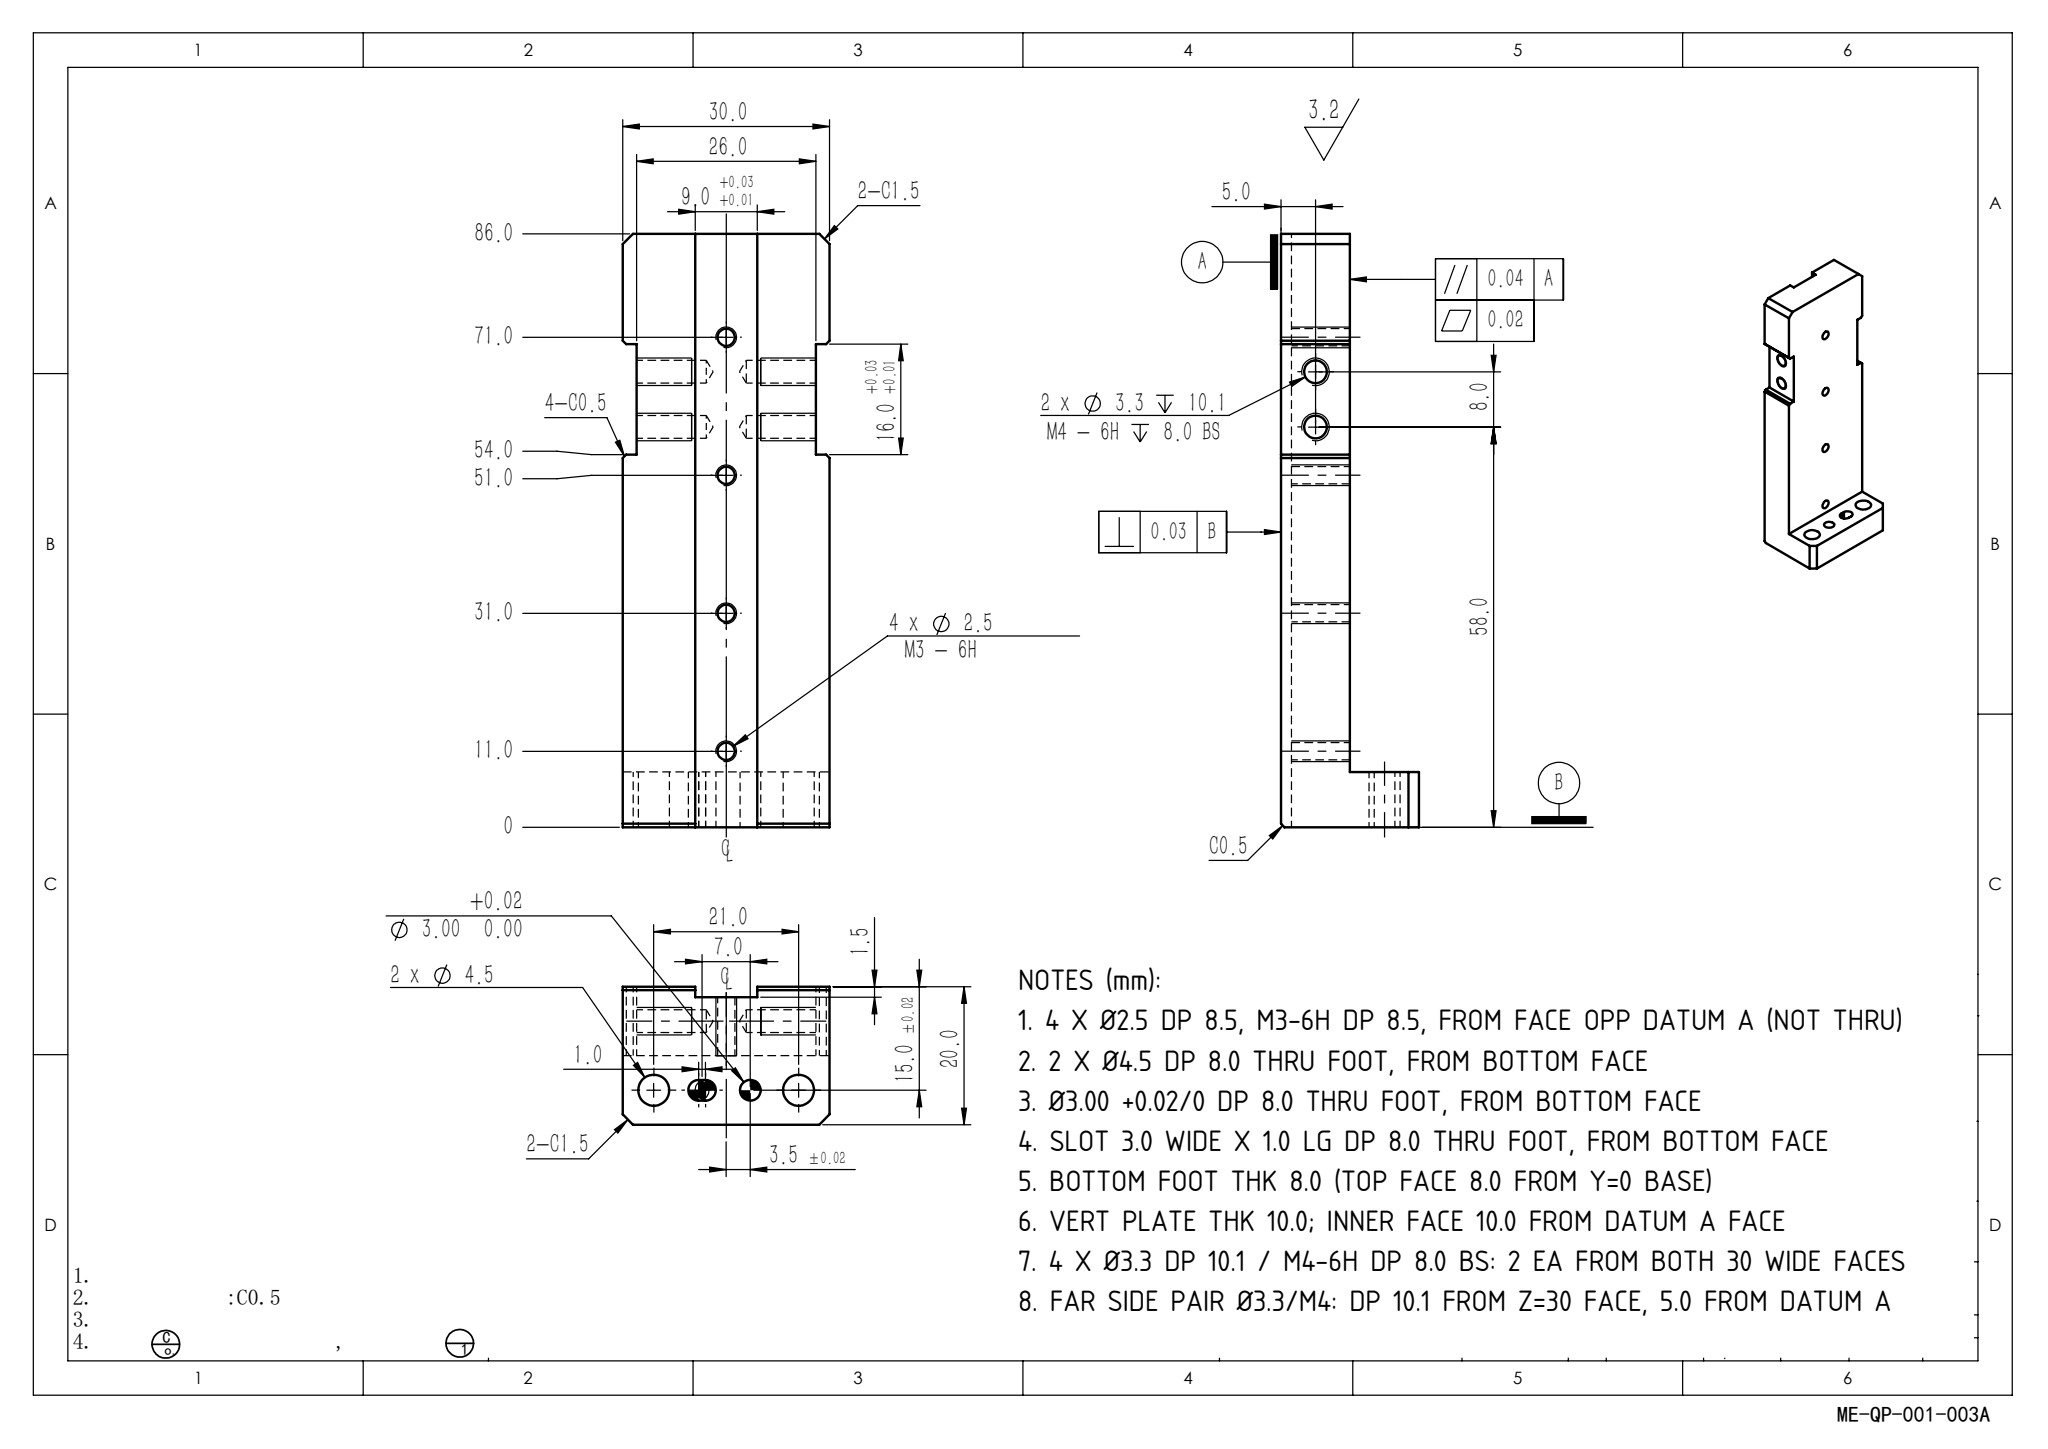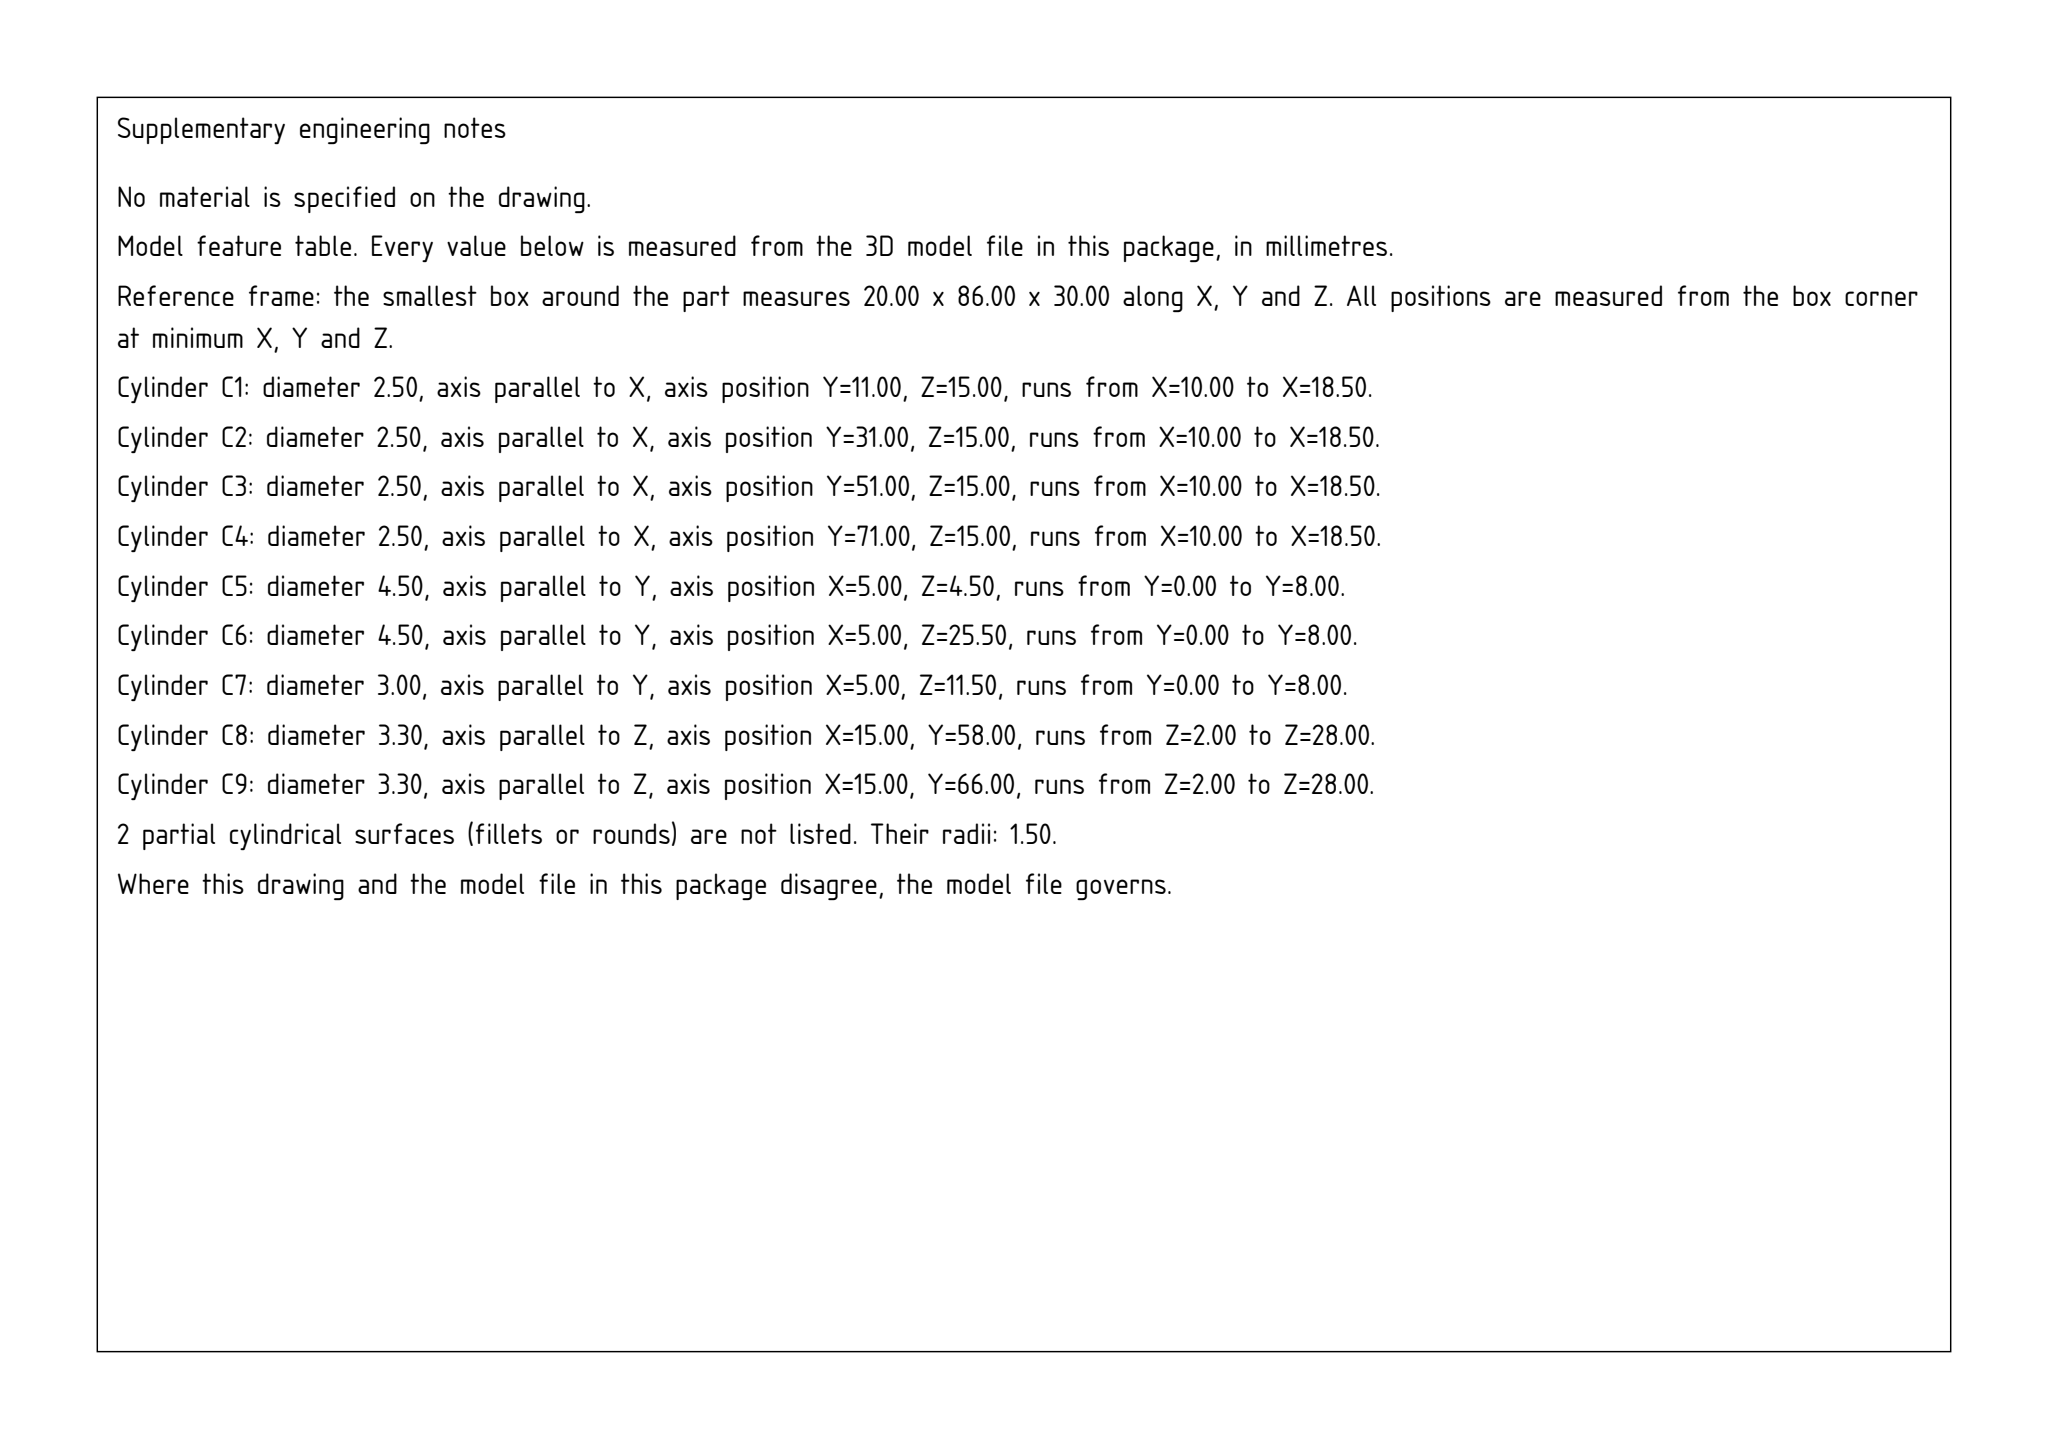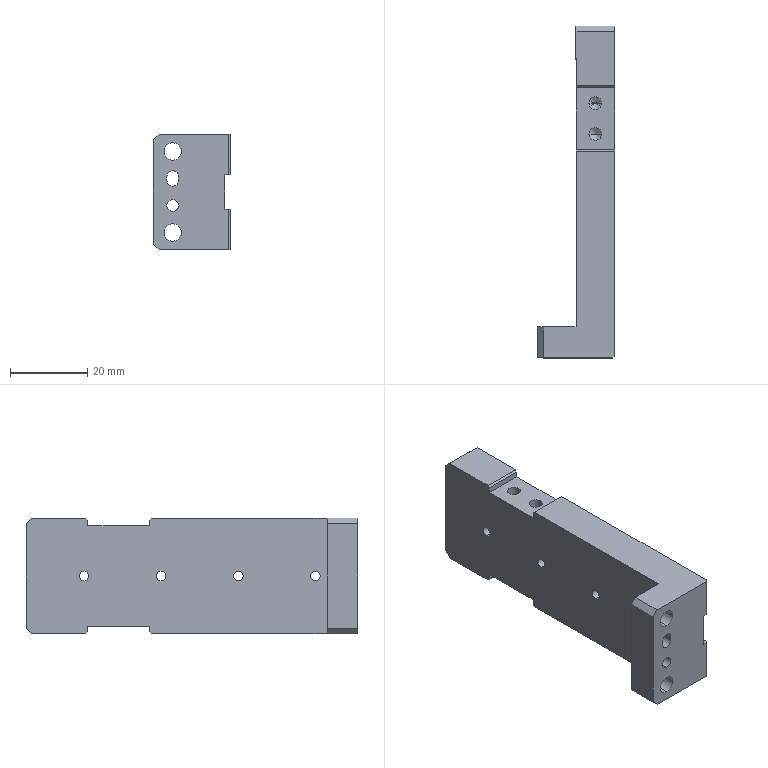Part | SolidWorks | mm | 1 solid | 64 faces | box 20 x 86 x 30 mm | volume 25436 mm3 | plane 32 | cylinder 24 | cone 8 | commonest cylinder face diameters 3.3 x8 2.5 x8 3 x4 4.5 x4
Drawing notes:
4 X Ø2.5 DP 8.5, M3-6H DP 8.5, FROM FACE OPP DATUM A (NOT THRU) | from the solid: cyl dia2.5 axis x len 8.5 at y=11/31/51/71, z=15; faces x=10.0 to x=18.5
2 X Ø4.5 DP 8.0 THRU FOOT, FROM BOTTOM FACE | from the solid: cyl dia4.5 axis y len 8.0 at x=5.0, z=4.5 & 25.5; foot face y=0 to 8.0
Ø3.00 +0.02/0 DP 8.0 THRU FOOT, FROM BOTTOM FACE | from the solid: cyl dia3.0 axis y len 8.0 at x=5.0, z=11.5
SLOT 3.0 WIDE X 1.0 LG DP 8.0 THRU FOOT, FROM BOTTOM FACE | from the solid: cyl dia3.0 axis y len 8.0 at z=18.0 & 19.0, x=5.0
BOTTOM FOOT THK 8.0 (TOP FACE 8.0 FROM Y=0 BASE) | from the solid: planes y=0.0 and y=8.0
VERT PLATE THK 10.0; INNER FACE 10.0 FROM DATUM A FACE | from the solid: planes x=20.0 (datum A) and x=10.0; overall 20.0
4 X Ø3.3 DP 10.1 / M4-6H DP 8.0 BS: 2 EA FROM BOTH 30 WIDE FACES | from the solid: dia3.3 axis z len 10.1 at (x=15, y=58) & (x=15, y=66), 4 off
FAR SIDE PAIR Ø3.3/M4: DP 10.1 FROM Z=30 FACE, 5.0 FROM DATUM A | from the solid: planes z=0 & z=30; holes x=15 (5.0 from x=20 datum A), len 10.1 each side
build123d program:
from build123d import *

# Parameters (mm, degrees)
BOSS_EXTRUDE1_DEPTH                 = 15
F_4_5_4_5_DIAMETER_HOLE1_D          = 4.5
SKETCH6_W                           = 9
SKETCH6_H                           = 86
CUT_EXTRUDE1_DEPTH                  = 1.5
SIZE_MM_CLEARANCE_DOWEL_PIN_HOLE1_D = 3
CUT_EXTRUDE2_DEPTH                  = 82.908
M3_TAPPED_HOLE1_D                   = 2.5
CUT_EXTRUDE3_DEPTH                  = 90.56
CUT_EXTRUDE3_DEPTH_BACK             = 90.56
SKETCH18_W                          = 2
SKETCH18_H                          = 16
M4_TAPPED_HOLE1_D                   = 3.3
M4_TAPPED_HOLE1_DEPTH               = 10.1
M4_TAPPED_HOLE1_TIP                 = 0.9914
M4_TAPPED_HOLE2_D                   = 3.3
M4_TAPPED_HOLE2_DEPTH               = 10.1
M4_TAPPED_HOLE2_TIP                 = 0.9914
CHAMFER1_SIZE                       = 1.5
CHAMFER2_SIZE                       = 0.5
CHAMFER3_SIZE                       = 0.5


with BuildPart() as part:
    # Sketch1 → Boss-Extrude1 (new, symmetric)
    with BuildSketch(Plane.XY):
        Polygon((0, 0), (0, 86), (-10, 86), (-10, 8), (-20, 8), (-20, 0), align=None)
    extrude(amount=BOSS_EXTRUDE1_DEPTH, both=True)

    # 4.5 _4.5_ Diameter Hole1 (through all)
    with Locations(Plane(origin=(0, 8, 0), x_dir=(1, 0, 0), z_dir=(0, 1, 0))):
        with Locations((-15, 10.5), (-15, -10.5)):
            Hole(F_4_5_4_5_DIAMETER_HOLE1_D / 2)

    # Sketch6 → Cut-Extrude1 (cut)
    with BuildSketch(Plane(origin=(0, 0, 0), x_dir=(0, 0, -1), z_dir=(1, 0, 0))):
        with Locations((0, 43)):
            Rectangle(SKETCH6_W, SKETCH6_H)
    extrude(amount=-CUT_EXTRUDE1_DEPTH, mode=Mode.SUBTRACT)

    # Size mm Clearance Dowel Pin Hole1 (through all)
    with Locations(Plane(origin=(0, 8, 0), x_dir=(1, 0, 0), z_dir=(0, 1, 0))):
        with Locations((-15, 3.5), (-15, -3.5)):
            Hole(SIZE_MM_CLEARANCE_DOWEL_PIN_HOLE1_D / 2)

    # Sketch15 → Cut-Extrude2 (cut, through all)
    with BuildSketch(Plane(origin=(0, 8, 0), x_dir=(1, 0, 0), z_dir=(0, 1, 0))):
        with BuildLine():
            Line((-13.5, -3), (-13.5, -4))
            ThreePointArc((-13.5, -4), (-15, -5.5), (-16.5, -4))
            Line((-16.5, -4), (-16.5, -3))
            ThreePointArc((-16.5, -3), (-15, -1.5), (-13.5, -3))
        make_face()
    extrude(amount=-CUT_EXTRUDE2_DEPTH, mode=Mode.SUBTRACT)

    # M3 Tapped Hole1 (through all)
    with Locations(Plane(origin=(-1.5, 0, 0), x_dir=(0, 0, -1), z_dir=(1, 0, 0))):
        with Locations((0, 71), (0, 51), (0, 31), (0, 11)):
            Hole(M3_TAPPED_HOLE1_D / 2)

    # Sketch18 → Cut-Extrude3 (cut, two sides: drawn at the far end of the back side and taken through both)
    with BuildSketch(Plane(origin=(0, 0, 0), x_dir=(0, 0, -1), z_dir=(1, 0, 0)).offset(-CUT_EXTRUDE3_DEPTH_BACK)):
        with Locations((-14, 62)):
            Rectangle(SKETCH18_W, SKETCH18_H)
        with Locations((14, 62)):
            Rectangle(SKETCH18_W, SKETCH18_H)
    extrude(amount=CUT_EXTRUDE3_DEPTH + CUT_EXTRUDE3_DEPTH_BACK, mode=Mode.SUBTRACT)

    # M4 Tapped Hole1
    with Locations(Plane.XY.offset(13)):
        with Locations((-5, 66), (-5, 58)):
            Hole(M4_TAPPED_HOLE1_D / 2, depth=M4_TAPPED_HOLE1_DEPTH)
            with Locations((0, 0, -(M4_TAPPED_HOLE1_DEPTH + M4_TAPPED_HOLE1_TIP / 2))):  # 118° drill point
                Cone(0, M4_TAPPED_HOLE1_D / 2, M4_TAPPED_HOLE1_TIP, mode=Mode.SUBTRACT)

    # M4 Tapped Hole2
    with Locations(Plane(origin=(0, 0, -13), x_dir=(-1, 0, 0), z_dir=(0, 0, -1))):
        with Locations((5, 66), (5, 58)):
            Hole(M4_TAPPED_HOLE2_D / 2, depth=M4_TAPPED_HOLE2_DEPTH)
            with Locations((0, 0, -(M4_TAPPED_HOLE2_DEPTH + M4_TAPPED_HOLE2_TIP / 2))):  # 118° drill point
                Cone(0, M4_TAPPED_HOLE2_D / 2, M4_TAPPED_HOLE2_TIP, mode=Mode.SUBTRACT)

    # Chamfer1
    chamfer1_edges = [part.edges().sort_by_distance(p)[0] for p in [
        (-5, 86, 15),
        (-20, 4, 15),
        (-20, 4, -15),
        (-5, 86, -15),
    ]]
    chamfer(chamfer1_edges, length=CHAMFER1_SIZE)

    # Chamfer2
    chamfer2_edges = [part.edges().sort_by_distance(p)[0] for p in [
        (0, 0, 9.75),
        (0, 0, -9.75),
    ]]
    chamfer(chamfer2_edges, length=CHAMFER2_SIZE)

    # Chamfer3
    chamfer3_edges = [part.edges().sort_by_distance(p)[0] for p in [
        (-5, 54, 15),
        (-5, 70, 15),
        (-5, 70, -15),
        (-5, 54, -15),
    ]]
    chamfer(chamfer3_edges, length=CHAMFER3_SIZE)


solid = part.part